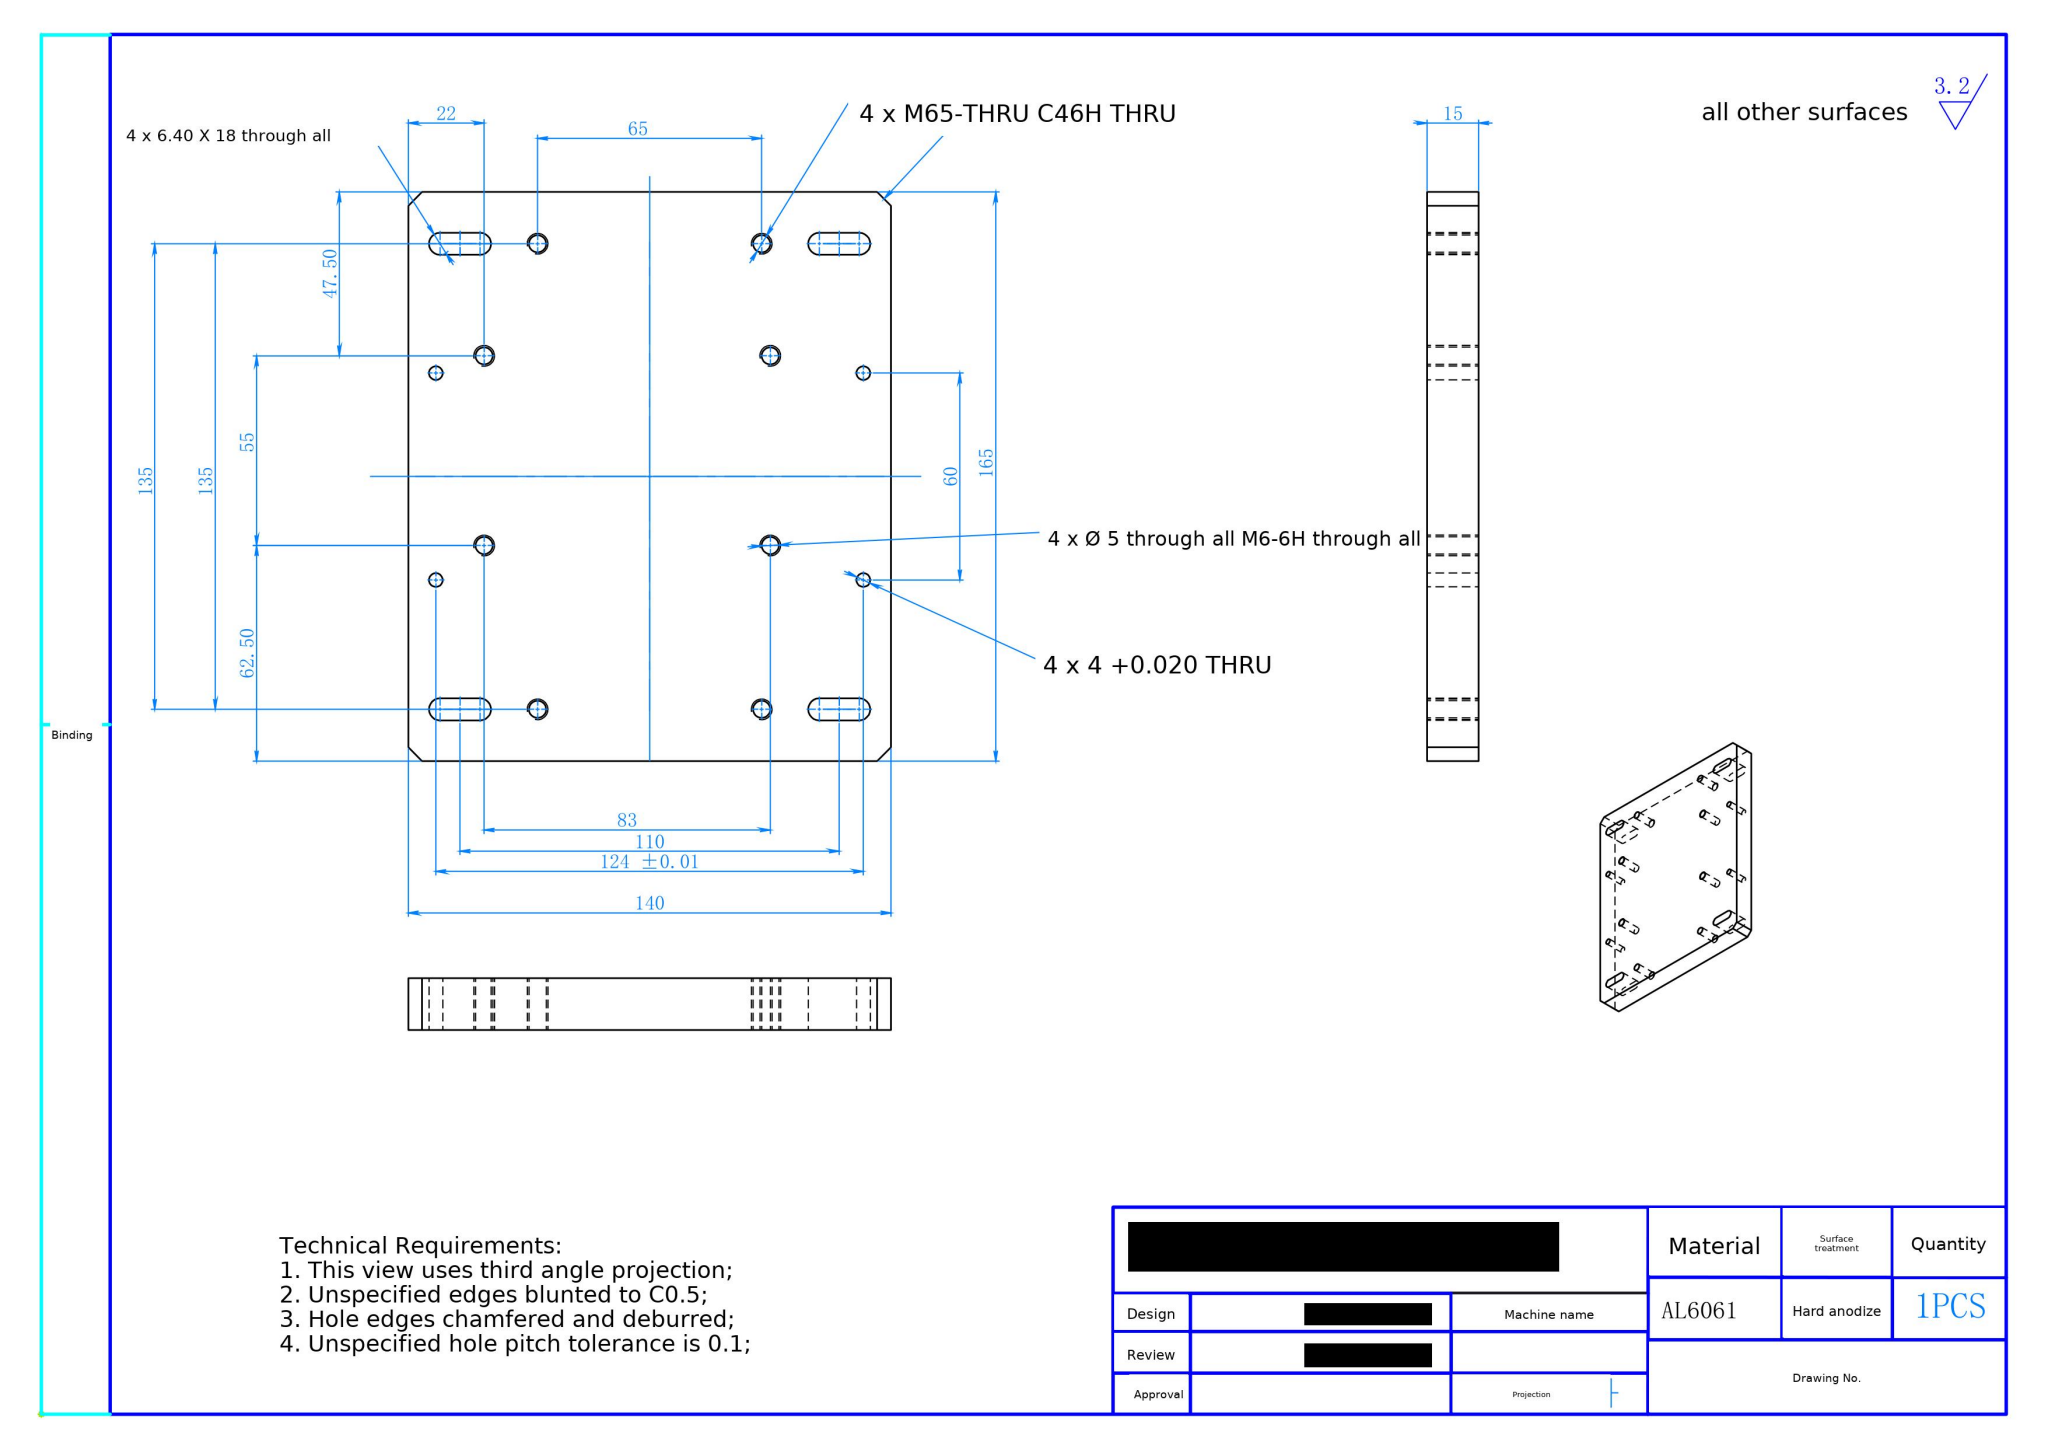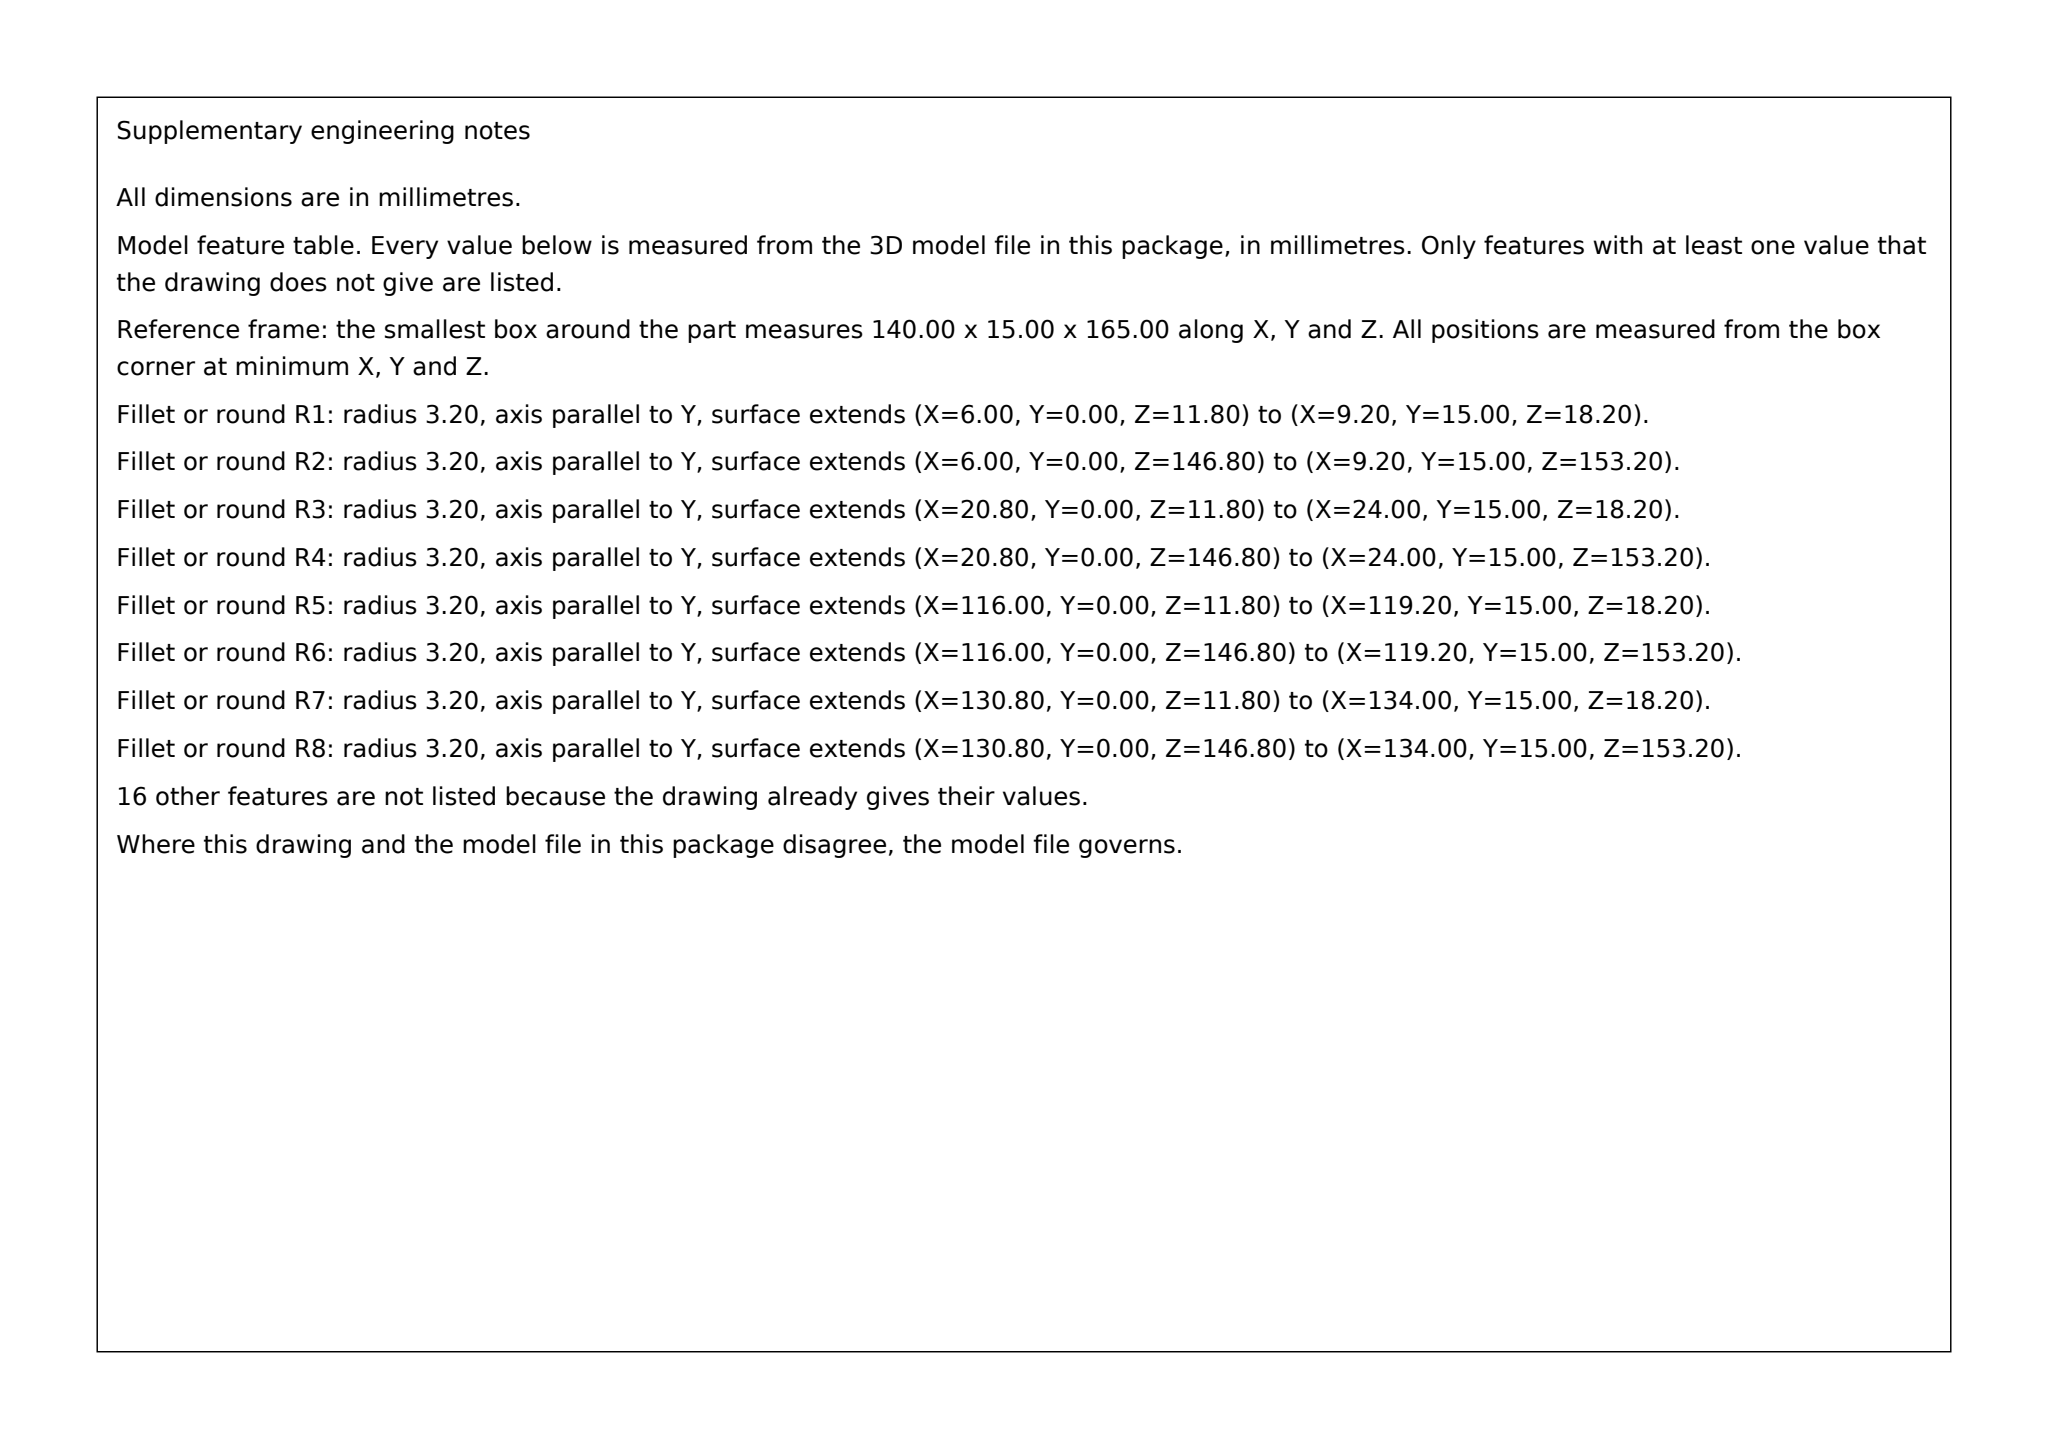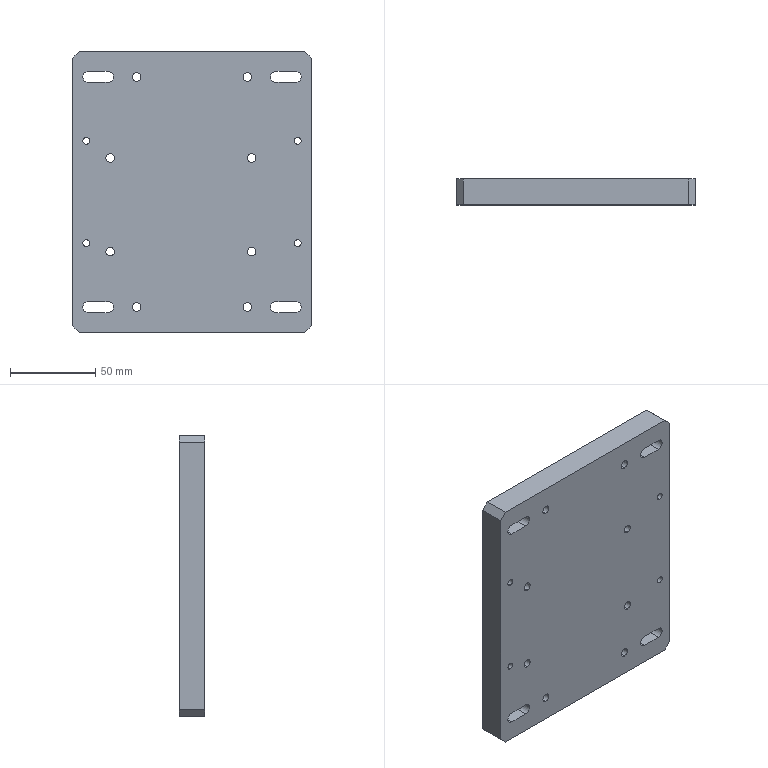Part | SolidWorks | mm | material AL6061 | 1 solid | 50 faces | box 140 x 15 x 165 mm | volume 336525 mm3 | cylinder 32 | plane 18 | commonest cylinder face diameters 5 x16 4 x8 6.4 x8